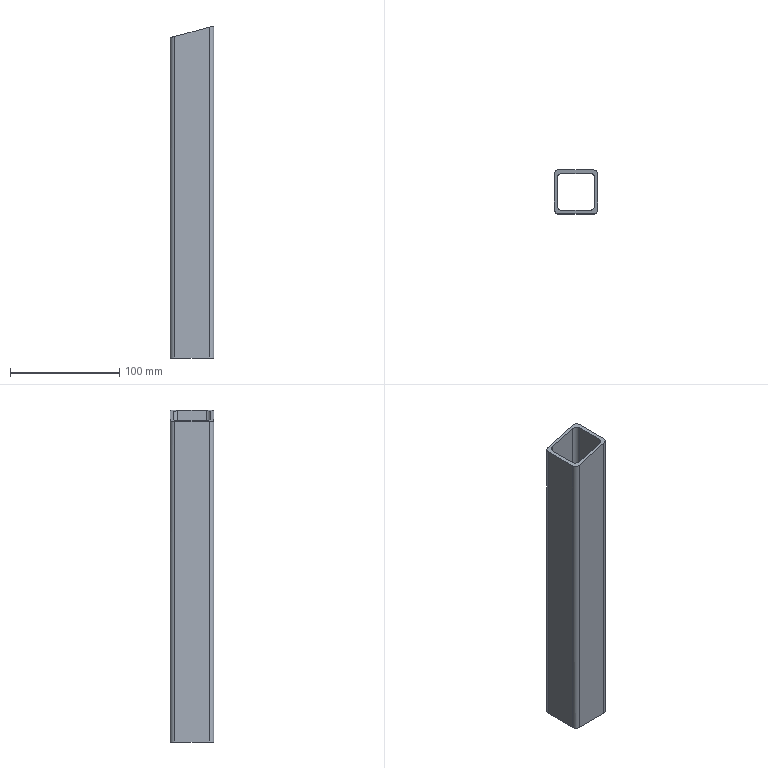Component | NX | SLANT_VERT_ROD_3_2 | 1 solid | 18 faces | volume 132665 mm3 | plane 10 | cylinder 8 | commonest cylinder face diameters 8 x8